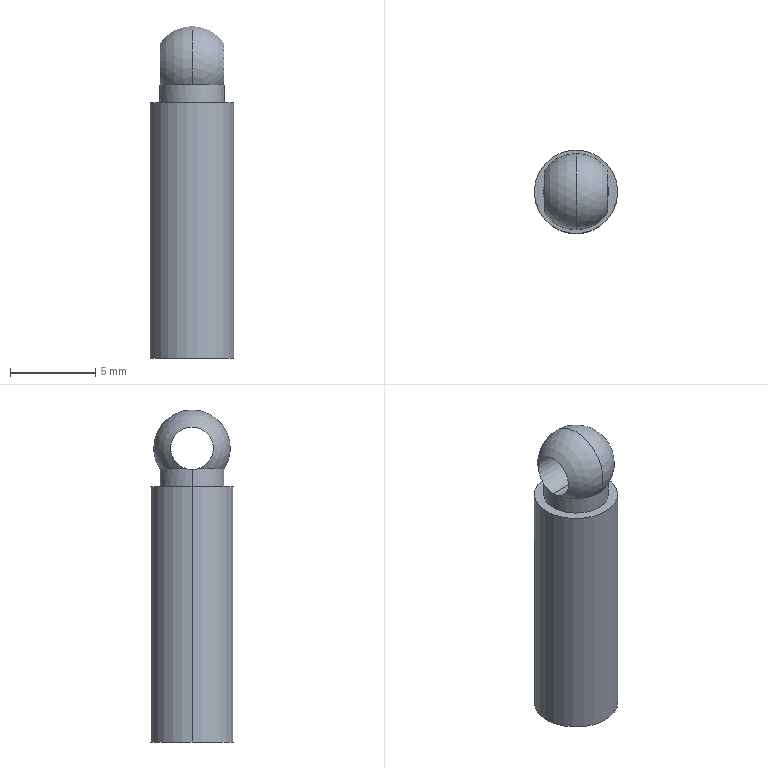Component | SolidWorks | RoundHead-3 | 1 solid | 14 faces | box 4.9 x 4.9 x 19.5 mm | volume 168 mm3 | cylinder 8 | cone 2 | sphere 2 | plane 2 | commonest cylinder face diameters 3.5 x2 2.5 x2 3.8 x2 4.9 x2
build123d program:
from build123d import *

# Parameters (mm, degrees)
SKETCH1_R                      = 2.45
EXTRUDE1_DEPTH                 = 15
SKETCH2_R                      = 1.9
EXTRUDE2_DEPTH                 = 1.5
CUT_EXTRUDE1_DEPTH             = 20.805
CUT_EXTRUDE1_DEPTH_BACK        = 20.805
SKETCH4_R                      = 1.25
F_3_5_3_5_DIAMETER_HOLE1_D     = 3.5
F_3_5_3_5_DIAMETER_HOLE1_DEPTH = 15
F_3_5_3_5_DIAMETER_HOLE1_TIP   = 1.052


with BuildPart() as part:
    # Sketch1 → Extrude1 (new body)
    with BuildSketch(Plane(origin=(0, 0, 0), x_dir=(0, 0, -1), z_dir=(1, 0, 0))):
        Circle(SKETCH1_R)
    extrude(amount=EXTRUDE1_DEPTH)

    # Sketch2 → Extrude2 (add)
    with BuildSketch(Plane(origin=(15, 0, 0), x_dir=(0, 0, -1), z_dir=(1, 0, 0))):
        Circle(SKETCH2_R)
    extrude(amount=EXTRUDE2_DEPTH)

    # Sketch3 → Revolve1 (revolve)
    with BuildSketch(Plane.XY):
        with BuildLine():
            Line((15, 0), (19.5, 0))
            ThreePointArc((19.5, 0), (17.25, -2.25), (15, 0))
        make_face()
    revolve(axis=Axis((15, 0, 0), (1, 0, 0)))

    # Sketch4 → Cut-Extrude1 (cut, two sides: drawn at the far end of the back side and taken through both)
    with BuildSketch(Plane.XY.offset(-CUT_EXTRUDE1_DEPTH_BACK)):
        with Locations(Location((17.25, 0, 0), (0, 0, 164.613))):
            Circle(SKETCH4_R)
    extrude(amount=CUT_EXTRUDE1_DEPTH + CUT_EXTRUDE1_DEPTH_BACK, mode=Mode.SUBTRACT)

    # 3.5 _3.5_ Diameter Hole1
    with Locations(Plane.ZY):
        with Locations((0, 0)):
            Hole(F_3_5_3_5_DIAMETER_HOLE1_D / 2, depth=F_3_5_3_5_DIAMETER_HOLE1_DEPTH)
            with Locations((0, 0, -(F_3_5_3_5_DIAMETER_HOLE1_DEPTH + F_3_5_3_5_DIAMETER_HOLE1_TIP / 2))):  # 118° drill point
                Cone(0, F_3_5_3_5_DIAMETER_HOLE1_D / 2, F_3_5_3_5_DIAMETER_HOLE1_TIP, mode=Mode.SUBTRACT)


solid = part.part

# Placed as in the assembly
solid = solid.moved(Location((12.867, 79.622, -192.387), (0, -90, 0)))
STEP:
#1=CARTESIAN_POINT('',(0.5755,3.135,-6.984));
#2=VERTEX_POINT('',#1);
#3=CARTESIAN_POINT('',(0.4377,3.135,-6.984));
#4=VERTEX_POINT('',#3);
#5=CARTESIAN_POINT('',(0.5066,3.135,-6.984));
#6=DIRECTION('',(-0.,0.,-1.));
#7=DIRECTION('',(-1.,0.,0.));
#8=AXIS2_PLACEMENT_3D('',#5,#6,#7);
#9=CIRCLE('',#8,0.0689);
#10=EDGE_CURVE('',#2,#4,#9,.T.);
#11=ORIENTED_EDGE('',*,*,#10,.F.);
#12=CARTESIAN_POINT('',(0.5755,3.135,-7.574));
#13=VERTEX_POINT('',#12);
#14=CARTESIAN_POINT('',(0.5755,3.135,-7.574));
#15=DIRECTION('',(-0.,0.,-1.));
#16=VECTOR('',#15,39.37);
#17=LINE('',#14,#16);
#18=EDGE_CURVE('',#2,#13,#17,.T.);
#19=ORIENTED_EDGE('',*,*,#18,.T.);
#20=CARTESIAN_POINT('',(0.4377,3.135,-7.574));
#21=VERTEX_POINT('',#20);
#22=CARTESIAN_POINT('',(0.5066,3.135,-7.574));
#23=DIRECTION('',(-0.,0.,-1.));
#24=DIRECTION('',(-1.,0.,0.));
#25=AXIS2_PLACEMENT_3D('',#22,#23,#24);
#26=CIRCLE('',#25,0.0689);
#27=EDGE_CURVE('',#13,#21,#26,.T.);
#28=ORIENTED_EDGE('',*,*,#27,.T.);
#29=CARTESIAN_POINT('',(0.4377,3.135,-7.574));
#30=DIRECTION('',(-0.,0.,-1.));
#31=VECTOR('',#30,39.37);
#32=LINE('',#29,#31);
#33=EDGE_CURVE('',#4,#21,#32,.T.);
#34=ORIENTED_EDGE('',*,*,#33,.F.);
#35=EDGE_LOOP('',(#11,#19,#28,#34));
#36=FACE_OUTER_BOUND('',#35,.T.);
#37=CARTESIAN_POINT('',(0.5066,3.135,-7.574));
#38=DIRECTION('',(-0.,0.,-1.));
#39=DIRECTION('',(-1.,0.,0.));
#40=AXIS2_PLACEMENT_3D('',#37,#38,#39);
#41=CYLINDRICAL_SURFACE('',#40,0.0689);
#42=ADVANCED_FACE('',(#36),#41,.F.);
#43=CARTESIAN_POINT('',(0.5099,3.135,-6.944));
#44=VERTEX_POINT('',#43);
#45=CARTESIAN_POINT('',(0.5032,3.135,-6.944));
#46=VERTEX_POINT('',#45);
#47=CARTESIAN_POINT('',(0.5099,3.135,-6.944));
#48=CARTESIAN_POINT('',(0.5099,3.134,-6.944));
#49=CARTESIAN_POINT('',(0.5099,3.134,-6.944));
#50=CARTESIAN_POINT('',(0.5098,3.134,-6.944));
#51=CARTESIAN_POINT('',(0.5098,3.134,-6.944));
#52=CARTESIAN_POINT('',(0.5096,3.133,-6.944));
#53=CARTESIAN_POINT('',(0.5094,3.133,-6.944));
#54=CARTESIAN_POINT('',(0.5092,3.133,-6.944));
#55=CARTESIAN_POINT('',(0.509,3.132,-6.944));
#56=CARTESIAN_POINT('',(0.5087,3.132,-6.944));
#57=CARTESIAN_POINT('',(0.5084,3.132,-6.944));
#58=CARTESIAN_POINT('',(0.5081,3.132,-6.944));
#59=CARTESIAN_POINT('',(0.5078,3.132,-6.944));
#60=CARTESIAN_POINT('',(0.5075,3.132,-6.944));
#61=CARTESIAN_POINT('',(0.5073,3.132,-6.944));
#62=CARTESIAN_POINT('',(0.5071,3.132,-6.944));
#63=CARTESIAN_POINT('',(0.5067,3.132,-6.944));
#64=CARTESIAN_POINT('',(0.5063,3.132,-6.944));
#65=CARTESIAN_POINT('',(0.5059,3.132,-6.944));
#66=CARTESIAN_POINT('',(0.5055,3.132,-6.944));
#67=CARTESIAN_POINT('',(0.5051,3.132,-6.944));
#68=CARTESIAN_POINT('',(0.5048,3.132,-6.944));
#69=CARTESIAN_POINT('',(0.5044,3.132,-6.944));
#70=CARTESIAN_POINT('',(0.5041,3.132,-6.944));
#71=CARTESIAN_POINT('',(0.5039,3.133,-6.944));
#72=CARTESIAN_POINT('',(0.5037,3.133,-6.944));
#73=CARTESIAN_POINT('',(0.5035,3.133,-6.944));
#74=CARTESIAN_POINT('',(0.5034,3.134,-6.944));
#75=CARTESIAN_POINT('',(0.5032,3.134,-6.944));
#76=CARTESIAN_POINT('',(0.5032,3.134,-6.944));
#77=CARTESIAN_POINT('',(0.5032,3.135,-6.944));
#78=B_SPLINE_CURVE_WITH_KNOTS('',3,(#47,#48,#49,#50,#51,#52,#53,#54,#55,#56,#57,#58,#59,#60,#61,#62,#63,#64,#65,#66,#67,#68,#69,#70,#71,#72,#73,#74,#75,#76,#77),.UNSPECIFIED.,.F.,.F.,(4,3,3,3,3,3,3,3,3,3,4),(0.0004044,0.0004243,0.00045,0.0004765,0.0005043,0.0005219,0.000552,0.0005822,0.0006119,0.0006404,0.0006654),.UNSPECIFIED.);
#79=EDGE_CURVE('',#44,#46,#78,.T.);
#80=ORIENTED_EDGE('',*,*,#79,.F.);
#81=CARTESIAN_POINT('',(0.5755,3.135,-6.984));
#82=DIRECTION('',(0.8572,0.,-0.515));
#83=VECTOR('',#82,39.37);
#84=LINE('',#81,#83);
#85=EDGE_CURVE('',#44,#2,#84,.T.);
#86=ORIENTED_EDGE('',*,*,#85,.T.);
#87=ORIENTED_EDGE('',*,*,#10,.T.);
#88=CARTESIAN_POINT('',(0.4377,3.135,-6.984));
#89=DIRECTION('',(-0.8572,0.,-0.515));
#90=VECTOR('',#89,39.37);
#91=LINE('',#88,#90);
#92=EDGE_CURVE('',#46,#4,#91,.T.);
#93=ORIENTED_EDGE('',*,*,#92,.F.);
#94=EDGE_LOOP('',(#80,#86,#87,#93));
#95=FACE_OUTER_BOUND('',#94,.T.);
#96=CARTESIAN_POINT('',(0.5066,3.135,-6.984));
#97=DIRECTION('',(-0.,0.,-1.));
#98=DIRECTION('',(-1.,0.,0.));
#99=AXIS2_PLACEMENT_3D('',#96,#97,#98);
#100=CONICAL_SURFACE('',#99,0.0689,1.03);
#101=ADVANCED_FACE('',(#95),#100,.F.);
#102=CARTESIAN_POINT('',(0.5814,3.135,-6.944));
#103=VERTEX_POINT('',#102);
#104=CARTESIAN_POINT('',(0.5802,3.122,-6.943));
#105=VERTEX_POINT('',#104);
#106=CARTESIAN_POINT('',(0.5814,3.135,-6.944));
#107=CARTESIAN_POINT('',(0.5814,3.13,-6.944));
#108=CARTESIAN_POINT('',(0.581,3.126,-6.944));
#109=CARTESIAN_POINT('',(0.5802,3.122,-6.943));
#110=B_SPLINE_CURVE_WITH_KNOTS('',3,(#106,#107,#108,#109),.UNSPECIFIED.,.F.,.F.,(4,4),(0.0003359,0.0006708),.UNSPECIFIED.);
#111=EDGE_CURVE('',#103,#105,#110,.T.);
#112=ORIENTED_EDGE('',*,*,#111,.F.);
#113=CARTESIAN_POINT('',(0.603,3.135,-6.944));
#114=DIRECTION('',(-1.,0.,0.));
#115=VECTOR('',#114,39.37);
#116=LINE('',#113,#115);
#117=EDGE_CURVE('',#103,#44,#116,.T.);
#118=ORIENTED_EDGE('',*,*,#117,.T.);
#119=ORIENTED_EDGE('',*,*,#79,.T.);
#120=CARTESIAN_POINT('',(0.4318,3.135,-6.944));
#121=VERTEX_POINT('',#120);
#122=CARTESIAN_POINT('',(0.603,3.135,-6.944));
#123=DIRECTION('',(-1.,0.,0.));
#124=VECTOR('',#123,39.37);
#125=LINE('',#122,#124);
#126=EDGE_CURVE('',#46,#121,#125,.T.);
#127=ORIENTED_EDGE('',*,*,#126,.T.);
#128=CARTESIAN_POINT('',(0.4329,3.122,-6.943));
#129=VERTEX_POINT('',#128);
#130=CARTESIAN_POINT('',(0.4329,3.122,-6.943));
#131=CARTESIAN_POINT('',(0.4322,3.126,-6.944));
#132=CARTESIAN_POINT('',(0.4318,3.13,-6.944));
#133=CARTESIAN_POINT('',(0.4318,3.135,-6.944));
#134=B_SPLINE_CURVE_WITH_KNOTS('',3,(#130,#131,#132,#133),.UNSPECIFIED.,.F.,.F.,(4,4),(0.,0.0003359),.UNSPECIFIED.);
#135=EDGE_CURVE('',#129,#121,#134,.T.);
#136=ORIENTED_EDGE('',*,*,#135,.F.);
#137=CARTESIAN_POINT('',(0.4329,3.135,-6.846));
#138=VERTEX_POINT('',#137);
#139=CARTESIAN_POINT('',(0.4329,3.135,-6.895));
#140=DIRECTION('',(-1.,0.,0.));
#141=DIRECTION('',(0.,-0.,-1.));
#142=AXIS2_PLACEMENT_3D('',#139,#140,#141);
#143=CIRCLE('',#142,0.04921);
#144=EDGE_CURVE('',#129,#138,#143,.T.);
#145=ORIENTED_EDGE('',*,*,#144,.T.);
#146=CARTESIAN_POINT('',(0.5802,3.135,-6.846));
#147=VERTEX_POINT('',#146);
#148=CARTESIAN_POINT('',(0.603,3.135,-6.846));
#149=DIRECTION('',(-1.,0.,0.));
#150=VECTOR('',#149,39.37);
#151=LINE('',#148,#150);
#152=EDGE_CURVE('',#147,#138,#151,.T.);
#153=ORIENTED_EDGE('',*,*,#152,.F.);
#154=CARTESIAN_POINT('',(0.5802,3.135,-6.895));
#155=DIRECTION('',(1.,0.,-0.));
#156=DIRECTION('',(0.,0.,1.));
#157=AXIS2_PLACEMENT_3D('',#154,#155,#156);
#158=CIRCLE('',#157,0.04921);
#159=EDGE_CURVE('',#147,#105,#158,.T.);
#160=ORIENTED_EDGE('',*,*,#159,.T.);
#161=EDGE_LOOP('',(#112,#118,#119,#127,#136,#145,#153,#160));
#162=FACE_OUTER_BOUND('',#161,.T.);
#163=CARTESIAN_POINT('',(0.603,3.135,-6.895));
#164=DIRECTION('',(-1.,0.,0.));
#165=DIRECTION('',(0.,0.,1.));
#166=AXIS2_PLACEMENT_3D('',#163,#164,#165);
#167=CYLINDRICAL_SURFACE('',#166,0.04921);
#168=ADVANCED_FACE('',(#162),#167,.F.);
#169=CARTESIAN_POINT('',(0.5066,3.135,-6.807));
#170=VERTEX_POINT('',#169);
#171=CARTESIAN_POINT('',(0.5066,3.06,-6.943));
#172=VERTEX_POINT('',#171);
#173=CARTESIAN_POINT('',(0.5066,3.135,-6.895));
#174=DIRECTION('',(1.,0.,-0.));
#175=DIRECTION('',(0.,0.,-1.));
#176=AXIS2_PLACEMENT_3D('',#173,#174,#175);
#177=CIRCLE('',#176,0.08858);
#178=EDGE_CURVE('',#170,#172,#177,.T.);
#179=ORIENTED_EDGE('',*,*,#178,.F.);
#180=CARTESIAN_POINT('',(0.5066,3.21,-6.943));
#181=VERTEX_POINT('',#180);
#182=CARTESIAN_POINT('',(0.5066,3.135,-6.895));
#183=DIRECTION('',(-1.,-0.,0.));
#184=DIRECTION('',(0.,-1.,0.));
#185=AXIS2_PLACEMENT_3D('',#182,#183,#184);
#186=CIRCLE('',#185,0.08858);
#187=EDGE_CURVE('',#170,#181,#186,.T.);
#188=ORIENTED_EDGE('',*,*,#187,.T.);
#189=CARTESIAN_POINT('',(0.4329,3.148,-6.943));
#190=VERTEX_POINT('',#189);
#191=CARTESIAN_POINT('',(0.5066,3.135,-6.943));
#192=DIRECTION('',(-0.,0.,-1.));
#193=DIRECTION('',(1.,0.,0.));
#194=AXIS2_PLACEMENT_3D('',#191,#192,#193);
#195=CIRCLE('',#194,0.0748);
#196=EDGE_CURVE('',#190,#181,#195,.T.);
#197=ORIENTED_EDGE('',*,*,#196,.F.);
#198=CARTESIAN_POINT('',(0.4329,3.135,-6.895));
#199=DIRECTION('',(-1.,0.,0.));
#200=DIRECTION('',(0.,-0.,-1.));
#201=AXIS2_PLACEMENT_3D('',#198,#199,#200);
#202=CIRCLE('',#201,0.04921);
#203=EDGE_CURVE('',#138,#190,#202,.T.);
#204=ORIENTED_EDGE('',*,*,#203,.F.);
#205=ORIENTED_EDGE('',*,*,#144,.F.);
#206=CARTESIAN_POINT('',(0.5066,3.135,-6.943));
#207=DIRECTION('',(-0.,0.,-1.));
#208=DIRECTION('',(1.,0.,0.));
#209=AXIS2_PLACEMENT_3D('',#206,#207,#208);
#210=CIRCLE('',#209,0.0748);
#211=EDGE_CURVE('',#172,#129,#210,.T.);
#212=ORIENTED_EDGE('',*,*,#211,.F.);
#213=EDGE_LOOP('',(#179,#188,#197,#204,#205,#212));
#214=FACE_OUTER_BOUND('',#213,.T.);
#215=CARTESIAN_POINT('',(0.5066,3.135,-6.895));
#216=DIRECTION('',(-1.,0.,0.));
#217=DIRECTION('',(0.,-1.,0.));
#218=AXIS2_PLACEMENT_3D('',#215,#216,#217);
#219=SPHERICAL_SURFACE('',#218,0.08858);
#220=ADVANCED_FACE('',(#214),#219,.T.);
#221=CARTESIAN_POINT('',(0.5802,3.148,-6.943));
#222=VERTEX_POINT('',#221);
#223=CARTESIAN_POINT('',(0.5802,3.148,-6.943));
#224=CARTESIAN_POINT('',(0.581,3.144,-6.944));
#225=CARTESIAN_POINT('',(0.5814,3.139,-6.944));
#226=CARTESIAN_POINT('',(0.5814,3.135,-6.944));
#227=B_SPLINE_CURVE_WITH_KNOTS('',3,(#223,#224,#225,#226),.UNSPECIFIED.,.F.,.F.,(4,4),(0.,0.0003359),.UNSPECIFIED.);
#228=EDGE_CURVE('',#222,#103,#227,.T.);
#229=ORIENTED_EDGE('',*,*,#228,.T.);
#230=CARTESIAN_POINT('',(0.5814,3.135,-6.984));
#231=VERTEX_POINT('',#230);
#232=CARTESIAN_POINT('',(0.5814,3.135,-6.925));
#233=DIRECTION('',(-0.,0.,-1.));
#234=VECTOR('',#233,39.37);
#235=LINE('',#232,#234);
#236=EDGE_CURVE('',#103,#231,#235,.T.);
#237=ORIENTED_EDGE('',*,*,#236,.T.);
#238=CARTESIAN_POINT('',(0.4318,3.135,-6.984));
#239=VERTEX_POINT('',#238);
#240=CARTESIAN_POINT('',(0.5066,3.135,-6.984));
#241=DIRECTION('',(0.,0.,1.));
#242=DIRECTION('',(1.,0.,0.));
#243=AXIS2_PLACEMENT_3D('',#240,#241,#242);
#244=CIRCLE('',#243,0.0748);
#245=EDGE_CURVE('',#231,#239,#244,.T.);
#246=ORIENTED_EDGE('',*,*,#245,.T.);
#247=CARTESIAN_POINT('',(0.4318,3.135,-6.925));
#248=DIRECTION('',(-0.,0.,-1.));
#249=VECTOR('',#248,39.37);
#250=LINE('',#247,#249);
#251=EDGE_CURVE('',#121,#239,#250,.T.);
#252=ORIENTED_EDGE('',*,*,#251,.F.);
#253=CARTESIAN_POINT('',(0.4318,3.135,-6.944));
#254=CARTESIAN_POINT('',(0.4318,3.139,-6.944));
#255=CARTESIAN_POINT('',(0.4322,3.144,-6.944));
#256=CARTESIAN_POINT('',(0.4329,3.148,-6.943));
#257=B_SPLINE_CURVE_WITH_KNOTS('',3,(#253,#254,#255,#256),.UNSPECIFIED.,.F.,.F.,(4,4),(0.0003359,0.0006708),.UNSPECIFIED.);
#258=EDGE_CURVE('',#121,#190,#257,.T.);
#259=ORIENTED_EDGE('',*,*,#258,.T.);
#260=ORIENTED_EDGE('',*,*,#196,.T.);
#261=CARTESIAN_POINT('',(0.5066,3.135,-6.943));
#262=DIRECTION('',(-0.,0.,-1.));
#263=DIRECTION('',(1.,0.,0.));
#264=AXIS2_PLACEMENT_3D('',#261,#262,#263);
#265=CIRCLE('',#264,0.0748);
#266=EDGE_CURVE('',#181,#222,#265,.T.);
#267=ORIENTED_EDGE('',*,*,#266,.T.);
#268=EDGE_LOOP('',(#229,#237,#246,#252,#259,#260,#267));
#269=FACE_OUTER_BOUND('',#268,.T.);
#270=CARTESIAN_POINT('',(0.5066,3.135,-6.925));
#271=DIRECTION('',(-0.,0.,-1.));
#272=DIRECTION('',(-1.,0.,0.));
#273=AXIS2_PLACEMENT_3D('',#270,#271,#272);
#274=CYLINDRICAL_SURFACE('',#273,0.0748);
#275=ADVANCED_FACE('',(#269),#274,.T.);
#276=CARTESIAN_POINT('',(0.603,3.135,-6.984));
#277=VERTEX_POINT('',#276);
#278=CARTESIAN_POINT('',(0.4101,3.135,-6.984));
#279=VERTEX_POINT('',#278);
#280=CARTESIAN_POINT('',(0.5066,3.135,-6.984));
#281=DIRECTION('',(0.,0.,1.));
#282=DIRECTION('',(1.,0.,0.));
#283=AXIS2_PLACEMENT_3D('',#280,#281,#282);
#284=CIRCLE('',#283,0.09646);
#285=EDGE_CURVE('',#277,#279,#284,.T.);
#286=ORIENTED_EDGE('',*,*,#285,.F.);
#287=CARTESIAN_POINT('',(0.603,3.135,-7.574));
#288=VERTEX_POINT('',#287);
#289=CARTESIAN_POINT('',(0.603,3.135,-6.984));
#290=DIRECTION('',(-0.,0.,-1.));
#291=VECTOR('',#290,39.37);
#292=LINE('',#289,#291);
#293=EDGE_CURVE('',#277,#288,#292,.T.);
#294=ORIENTED_EDGE('',*,*,#293,.T.);
#295=CARTESIAN_POINT('',(0.4101,3.135,-7.574));
#296=VERTEX_POINT('',#295);
#297=CARTESIAN_POINT('',(0.5066,3.135,-7.574));
#298=DIRECTION('',(0.,0.,1.));
#299=DIRECTION('',(1.,0.,0.));
#300=AXIS2_PLACEMENT_3D('',#297,#298,#299);
#301=CIRCLE('',#300,0.09646);
#302=EDGE_CURVE('',#288,#296,#301,.T.);
#303=ORIENTED_EDGE('',*,*,#302,.T.);
#304=CARTESIAN_POINT('',(0.4101,3.135,-6.984));
#305=DIRECTION('',(-0.,0.,-1.));
#306=VECTOR('',#305,39.37);
#307=LINE('',#304,#306);
#308=EDGE_CURVE('',#279,#296,#307,.T.);
#309=ORIENTED_EDGE('',*,*,#308,.F.);
#310=EDGE_LOOP('',(#286,#294,#303,#309));
#311=FACE_OUTER_BOUND('',#310,.T.);
#312=CARTESIAN_POINT('',(0.5066,3.135,-6.984));
#313=DIRECTION('',(-0.,0.,-1.));
#314=DIRECTION('',(-1.,0.,0.));
#315=AXIS2_PLACEMENT_3D('',#312,#313,#314);
#316=CYLINDRICAL_SURFACE('',#315,0.09646);
#317=ADVANCED_FACE('',(#311),#316,.T.);
#318=CARTESIAN_POINT('',(0.5066,3.135,-6.984));
#319=DIRECTION('',(0.,0.,1.));
#320=DIRECTION('',(1.,0.,0.));
#321=AXIS2_PLACEMENT_3D('',#318,#319,#320);
#322=CIRCLE('',#321,0.09646);
#323=EDGE_CURVE('',#279,#277,#322,.T.);
#324=ORIENTED_EDGE('',*,*,#323,.T.);
#325=ORIENTED_EDGE('',*,*,#285,.T.);
#326=EDGE_LOOP('',(#324,#325));
#327=FACE_OUTER_BOUND('',#326,.T.);
#328=CARTESIAN_POINT('',(0.5066,3.135,-6.984));
#329=DIRECTION('',(0.,0.,1.));
#330=DIRECTION('',(1.,0.,0.));
#331=AXIS2_PLACEMENT_3D('',#328,#329,#330);
#332=CIRCLE('',#331,0.0748);
#333=EDGE_CURVE('',#239,#231,#332,.T.);
#334=ORIENTED_EDGE('',*,*,#333,.F.);
#335=ORIENTED_EDGE('',*,*,#245,.F.);
#336=EDGE_LOOP('',(#334,#335));
#337=FACE_BOUND('',#336,.T.);
#338=CARTESIAN_POINT('',(0.5066,3.135,-6.984));
#339=DIRECTION('',(0.,0.,1.));
#340=DIRECTION('',(1.,0.,-0.));
#341=AXIS2_PLACEMENT_3D('',#338,#339,#340);
#342=PLANE('',#341);
#343=ADVANCED_FACE('',(#327,#337),#342,.T.);
#344=ORIENTED_EDGE('',*,*,#293,.F.);
#345=ORIENTED_EDGE('',*,*,#323,.F.);
#346=ORIENTED_EDGE('',*,*,#308,.T.);
#347=CARTESIAN_POINT('',(0.5066,3.135,-7.574));
#348=DIRECTION('',(0.,0.,1.));
#349=DIRECTION('',(1.,0.,0.));
#350=AXIS2_PLACEMENT_3D('',#347,#348,#349);
#351=CIRCLE('',#350,0.09646);
#352=EDGE_CURVE('',#296,#288,#351,.T.);
#353=ORIENTED_EDGE('',*,*,#352,.T.);
#354=EDGE_LOOP('',(#344,#345,#346,#353));
#355=FACE_OUTER_BOUND('',#354,.T.);
#356=CARTESIAN_POINT('',(0.5066,3.135,-6.984));
#357=DIRECTION('',(-0.,0.,-1.));
#358=DIRECTION('',(-1.,0.,0.));
#359=AXIS2_PLACEMENT_3D('',#356,#357,#358);
#360=CYLINDRICAL_SURFACE('',#359,0.09646);
#361=ADVANCED_FACE('',(#355),#360,.T.);
#362=CARTESIAN_POINT('',(0.5066,3.135,-7.574));
#363=DIRECTION('',(-0.,0.,-1.));
#364=DIRECTION('',(-1.,0.,0.));
#365=AXIS2_PLACEMENT_3D('',#362,#363,#364);
#366=CIRCLE('',#365,0.0689);
#367=EDGE_CURVE('',#21,#13,#366,.T.);
#368=ORIENTED_EDGE('',*,*,#367,.F.);
#369=ORIENTED_EDGE('',*,*,#27,.F.);
#370=EDGE_LOOP('',(#368,#369));
#371=FACE_BOUND('',#370,.T.);
#372=ORIENTED_EDGE('',*,*,#352,.F.);
#373=ORIENTED_EDGE('',*,*,#302,.F.);
#374=EDGE_LOOP('',(#372,#373));
#375=FACE_OUTER_BOUND('',#374,.T.);
#376=CARTESIAN_POINT('',(0.5066,3.135,-7.574));
#377=DIRECTION('',(0.,0.,1.));
#378=DIRECTION('',(1.,0.,-0.));
#379=AXIS2_PLACEMENT_3D('',#376,#377,#378);
#380=PLANE('',#379);
#381=ADVANCED_FACE('',(#371,#375),#380,.F.);
#382=ORIENTED_EDGE('',*,*,#236,.F.);
#383=ORIENTED_EDGE('',*,*,#111,.T.);
#384=CARTESIAN_POINT('',(0.5066,3.135,-6.943));
#385=DIRECTION('',(-0.,0.,-1.));
#386=DIRECTION('',(1.,0.,0.));
#387=AXIS2_PLACEMENT_3D('',#384,#385,#386);
#388=CIRCLE('',#387,0.0748);
#389=EDGE_CURVE('',#105,#172,#388,.T.);
#390=ORIENTED_EDGE('',*,*,#389,.T.);
#391=ORIENTED_EDGE('',*,*,#211,.T.);
#392=ORIENTED_EDGE('',*,*,#135,.T.);
#393=ORIENTED_EDGE('',*,*,#251,.T.);
#394=ORIENTED_EDGE('',*,*,#333,.T.);
#395=EDGE_LOOP('',(#382,#383,#390,#391,#392,#393,#394));
#396=FACE_OUTER_BOUND('',#395,.T.);
#397=CARTESIAN_POINT('',(0.5066,3.135,-6.925));
#398=DIRECTION('',(-0.,0.,-1.));
#399=DIRECTION('',(-1.,0.,0.));
#400=AXIS2_PLACEMENT_3D('',#397,#398,#399);
#401=CYLINDRICAL_SURFACE('',#400,0.0748);
#402=ADVANCED_FACE('',(#396),#401,.T.);
#403=ORIENTED_EDGE('',*,*,#187,.F.);
#404=ORIENTED_EDGE('',*,*,#178,.T.);
#405=ORIENTED_EDGE('',*,*,#389,.F.);
#406=ORIENTED_EDGE('',*,*,#159,.F.);
#407=CARTESIAN_POINT('',(0.5802,3.135,-6.895));
#408=DIRECTION('',(1.,0.,-0.));
#409=DIRECTION('',(0.,-0.,1.));
#410=AXIS2_PLACEMENT_3D('',#407,#408,#409);
#411=CIRCLE('',#410,0.04921);
#412=EDGE_CURVE('',#222,#147,#411,.T.);
#413=ORIENTED_EDGE('',*,*,#412,.F.);
#414=ORIENTED_EDGE('',*,*,#266,.F.);
#415=EDGE_LOOP('',(#403,#404,#405,#406,#413,#414));
#416=FACE_OUTER_BOUND('',#415,.T.);
#417=CARTESIAN_POINT('',(0.5066,3.135,-6.895));
#418=DIRECTION('',(-1.,0.,0.));
#419=DIRECTION('',(0.,-1.,0.));
#420=AXIS2_PLACEMENT_3D('',#417,#418,#419);
#421=SPHERICAL_SURFACE('',#420,0.08858);
#422=ADVANCED_FACE('',(#416),#421,.T.);
#423=ORIENTED_EDGE('',*,*,#117,.F.);
#424=ORIENTED_EDGE('',*,*,#228,.F.);
#425=ORIENTED_EDGE('',*,*,#412,.T.);
#426=ORIENTED_EDGE('',*,*,#152,.T.);
#427=ORIENTED_EDGE('',*,*,#203,.T.);
#428=ORIENTED_EDGE('',*,*,#258,.F.);
#429=ORIENTED_EDGE('',*,*,#126,.F.);
#430=CARTESIAN_POINT('',(0.5032,3.135,-6.944));
#431=CARTESIAN_POINT('',(0.5032,3.135,-6.944));
#432=CARTESIAN_POINT('',(0.5032,3.135,-6.944));
#433=CARTESIAN_POINT('',(0.5032,3.135,-6.944));
#434=CARTESIAN_POINT('',(0.5032,3.135,-6.944));
#435=CARTESIAN_POINT('',(0.5033,3.136,-6.944));
#436=CARTESIAN_POINT('',(0.5034,3.136,-6.944));
#437=CARTESIAN_POINT('',(0.5035,3.136,-6.944));
#438=CARTESIAN_POINT('',(0.5037,3.136,-6.944));
#439=CARTESIAN_POINT('',(0.5039,3.137,-6.944));
#440=CARTESIAN_POINT('',(0.5041,3.137,-6.944));
#441=CARTESIAN_POINT('',(0.5044,3.137,-6.944));
#442=CARTESIAN_POINT('',(0.5047,3.137,-6.944));
#443=CARTESIAN_POINT('',(0.505,3.138,-6.944));
#444=CARTESIAN_POINT('',(0.5054,3.138,-6.944));
#445=CARTESIAN_POINT('',(0.5057,3.138,-6.944));
#446=CARTESIAN_POINT('',(0.5061,3.138,-6.944));
#447=CARTESIAN_POINT('',(0.5065,3.138,-6.944));
#448=CARTESIAN_POINT('',(0.5069,3.138,-6.944));
#449=CARTESIAN_POINT('',(0.5073,3.138,-6.944));
#450=CARTESIAN_POINT('',(0.5077,3.138,-6.944));
#451=CARTESIAN_POINT('',(0.508,3.138,-6.944));
#452=CARTESIAN_POINT('',(0.5084,3.137,-6.944));
#453=CARTESIAN_POINT('',(0.5087,3.137,-6.944));
#454=CARTESIAN_POINT('',(0.509,3.137,-6.944));
#455=CARTESIAN_POINT('',(0.5093,3.137,-6.944));
#456=CARTESIAN_POINT('',(0.5095,3.136,-6.944));
#457=CARTESIAN_POINT('',(0.5097,3.136,-6.944));
#458=CARTESIAN_POINT('',(0.5098,3.136,-6.944));
#459=CARTESIAN_POINT('',(0.5099,3.135,-6.944));
#460=CARTESIAN_POINT('',(0.5099,3.135,-6.944));
#461=CARTESIAN_POINT('',(0.5099,3.135,-6.944));
#462=CARTESIAN_POINT('',(0.5099,3.135,-6.944));
#463=CARTESIAN_POINT('',(0.5099,3.135,-6.944));
#464=B_SPLINE_CURVE_WITH_KNOTS('',3,(#430,#431,#432,#433,#434,#435,#436,#437,#438,#439,#440,#441,#442,#443,#444,#445,#446,#447,#448,#449,#450,#451,#452,#453,#454,#455,#456,#457,#458,#459,#460,#461,#462,#463),.UNSPECIFIED.,.F.,.F.,(4,3,3,3,3,3,3,3,3,3,3,4),(0.0001435,0.0001454,0.0001713,0.0001972,0.0002241,0.0002523,0.0002818,0.000312,0.0003419,0.0003708,0.0003982,0.0004044),.UNSPECIFIED.);
#465=EDGE_CURVE('',#46,#44,#464,.T.);
#466=ORIENTED_EDGE('',*,*,#465,.T.);
#467=EDGE_LOOP('',(#423,#424,#425,#426,#427,#428,#429,#466));
#468=FACE_OUTER_BOUND('',#467,.T.);
#469=CARTESIAN_POINT('',(0.603,3.135,-6.895));
#470=DIRECTION('',(-1.,0.,0.));
#471=DIRECTION('',(0.,0.,1.));
#472=AXIS2_PLACEMENT_3D('',#469,#470,#471);
#473=CYLINDRICAL_SURFACE('',#472,0.04921);
#474=ADVANCED_FACE('',(#468),#473,.F.);
#475=ORIENTED_EDGE('',*,*,#85,.F.);
#476=ORIENTED_EDGE('',*,*,#465,.F.);
#477=ORIENTED_EDGE('',*,*,#92,.T.);
#478=CARTESIAN_POINT('',(0.5066,3.135,-6.984));
#479=DIRECTION('',(-0.,0.,-1.));
#480=DIRECTION('',(-1.,0.,0.));
#481=AXIS2_PLACEMENT_3D('',#478,#479,#480);
#482=CIRCLE('',#481,0.0689);
#483=EDGE_CURVE('',#4,#2,#482,.T.);
#484=ORIENTED_EDGE('',*,*,#483,.T.);
#485=EDGE_LOOP('',(#475,#476,#477,#484));
#486=FACE_OUTER_BOUND('',#485,.T.);
#487=CARTESIAN_POINT('',(0.5066,3.135,-6.984));
#488=DIRECTION('',(-0.,0.,-1.));
#489=DIRECTION('',(-1.,0.,0.));
#490=AXIS2_PLACEMENT_3D('',#487,#488,#489);
#491=CONICAL_SURFACE('',#490,0.0689,1.03);
#492=ADVANCED_FACE('',(#486),#491,.F.);
#493=ORIENTED_EDGE('',*,*,#18,.F.);
#494=ORIENTED_EDGE('',*,*,#483,.F.);
#495=ORIENTED_EDGE('',*,*,#33,.T.);
#496=ORIENTED_EDGE('',*,*,#367,.T.);
#497=EDGE_LOOP('',(#493,#494,#495,#496));
#498=FACE_OUTER_BOUND('',#497,.T.);
#499=CARTESIAN_POINT('',(0.5066,3.135,-7.574));
#500=DIRECTION('',(-0.,0.,-1.));
#501=DIRECTION('',(-1.,0.,0.));
#502=AXIS2_PLACEMENT_3D('',#499,#500,#501);
#503=CYLINDRICAL_SURFACE('',#502,0.0689);
#504=ADVANCED_FACE('',(#498),#503,.F.);
#505=CLOSED_SHELL('',(#42,#101,#168,#220,#275,#317,#343,#361,#381,#402,#422,#474,#492,#504));
#506=MANIFOLD_SOLID_BREP('',#505);
#507=CARTESIAN_POINT('',(0.,0.,0.));
#508=DIRECTION('',(0.,0.,1.));
#509=DIRECTION('',(1.,0.,0.));
#510=AXIS2_PLACEMENT_3D('',#507,#508,#509);
#511=(LENGTH_UNIT()NAMED_UNIT(*)SI_UNIT($,.METRE.));
#512=LENGTH_MEASURE_WITH_UNIT(LENGTH_MEASURE(0.0254),#511);
#513=DIMENSIONAL_EXPONENTS(1.,0.,0.,0.,0.,0.,0.);
#514=(CONVERSION_BASED_UNIT('',#512)LENGTH_UNIT()NAMED_UNIT(#513));
#515=UNCERTAINTY_MEASURE_WITH_UNIT(LENGTH_MEASURE(0.00001),#514,'','');
#516=(NAMED_UNIT(*)PLANE_ANGLE_UNIT()SI_UNIT($,.RADIAN.));
#517=(NAMED_UNIT(*)SI_UNIT($,.STERADIAN.)SOLID_ANGLE_UNIT());
#518=(GEOMETRIC_REPRESENTATION_CONTEXT(3)GLOBAL_UNCERTAINTY_ASSIGNED_CONTEXT((#515))GLOBAL_UNIT_ASSIGNED_CONTEXT((#514,#516,#517))REPRESENTATION_CONTEXT('',''));
#519=ADVANCED_BREP_SHAPE_REPRESENTATION('',(#506,#510),#518);
#520=COLOUR_RGB('',0.7922,0.8196,0.9333);
#521=FILL_AREA_STYLE_COLOUR('',#520);
#522=FILL_AREA_STYLE('',(#521));
#523=SURFACE_STYLE_FILL_AREA(#522);
#524=SURFACE_SIDE_STYLE('',(#523));
#525=SURFACE_STYLE_USAGE(.BOTH.,#524);
#526=PRESENTATION_STYLE_ASSIGNMENT((#525));
#527=STYLED_ITEM('',(#526),#506);
#528=PRESENTATION_LAYER_ASSIGNMENT('','',(#527));
#529=(LENGTH_UNIT()NAMED_UNIT(*)SI_UNIT($,.METRE.));
#530=LENGTH_MEASURE_WITH_UNIT(LENGTH_MEASURE(0.0254),#529);
#531=DIMENSIONAL_EXPONENTS(1.,0.,0.,0.,0.,0.,0.);
#532=(CONVERSION_BASED_UNIT('',#530)LENGTH_UNIT()NAMED_UNIT(#531));
#533=UNCERTAINTY_MEASURE_WITH_UNIT(LENGTH_MEASURE(0.00001),#532,'','');
#534=(NAMED_UNIT(*)PLANE_ANGLE_UNIT()SI_UNIT($,.RADIAN.));
#535=(NAMED_UNIT(*)SI_UNIT($,.STERADIAN.)SOLID_ANGLE_UNIT());
#536=(GEOMETRIC_REPRESENTATION_CONTEXT(3)GLOBAL_UNCERTAINTY_ASSIGNED_CONTEXT((#533))GLOBAL_UNIT_ASSIGNED_CONTEXT((#532,#534,#535))REPRESENTATION_CONTEXT('',''));
#537=MECHANICAL_DESIGN_GEOMETRIC_PRESENTATION_REPRESENTATION('',(#527),#536);